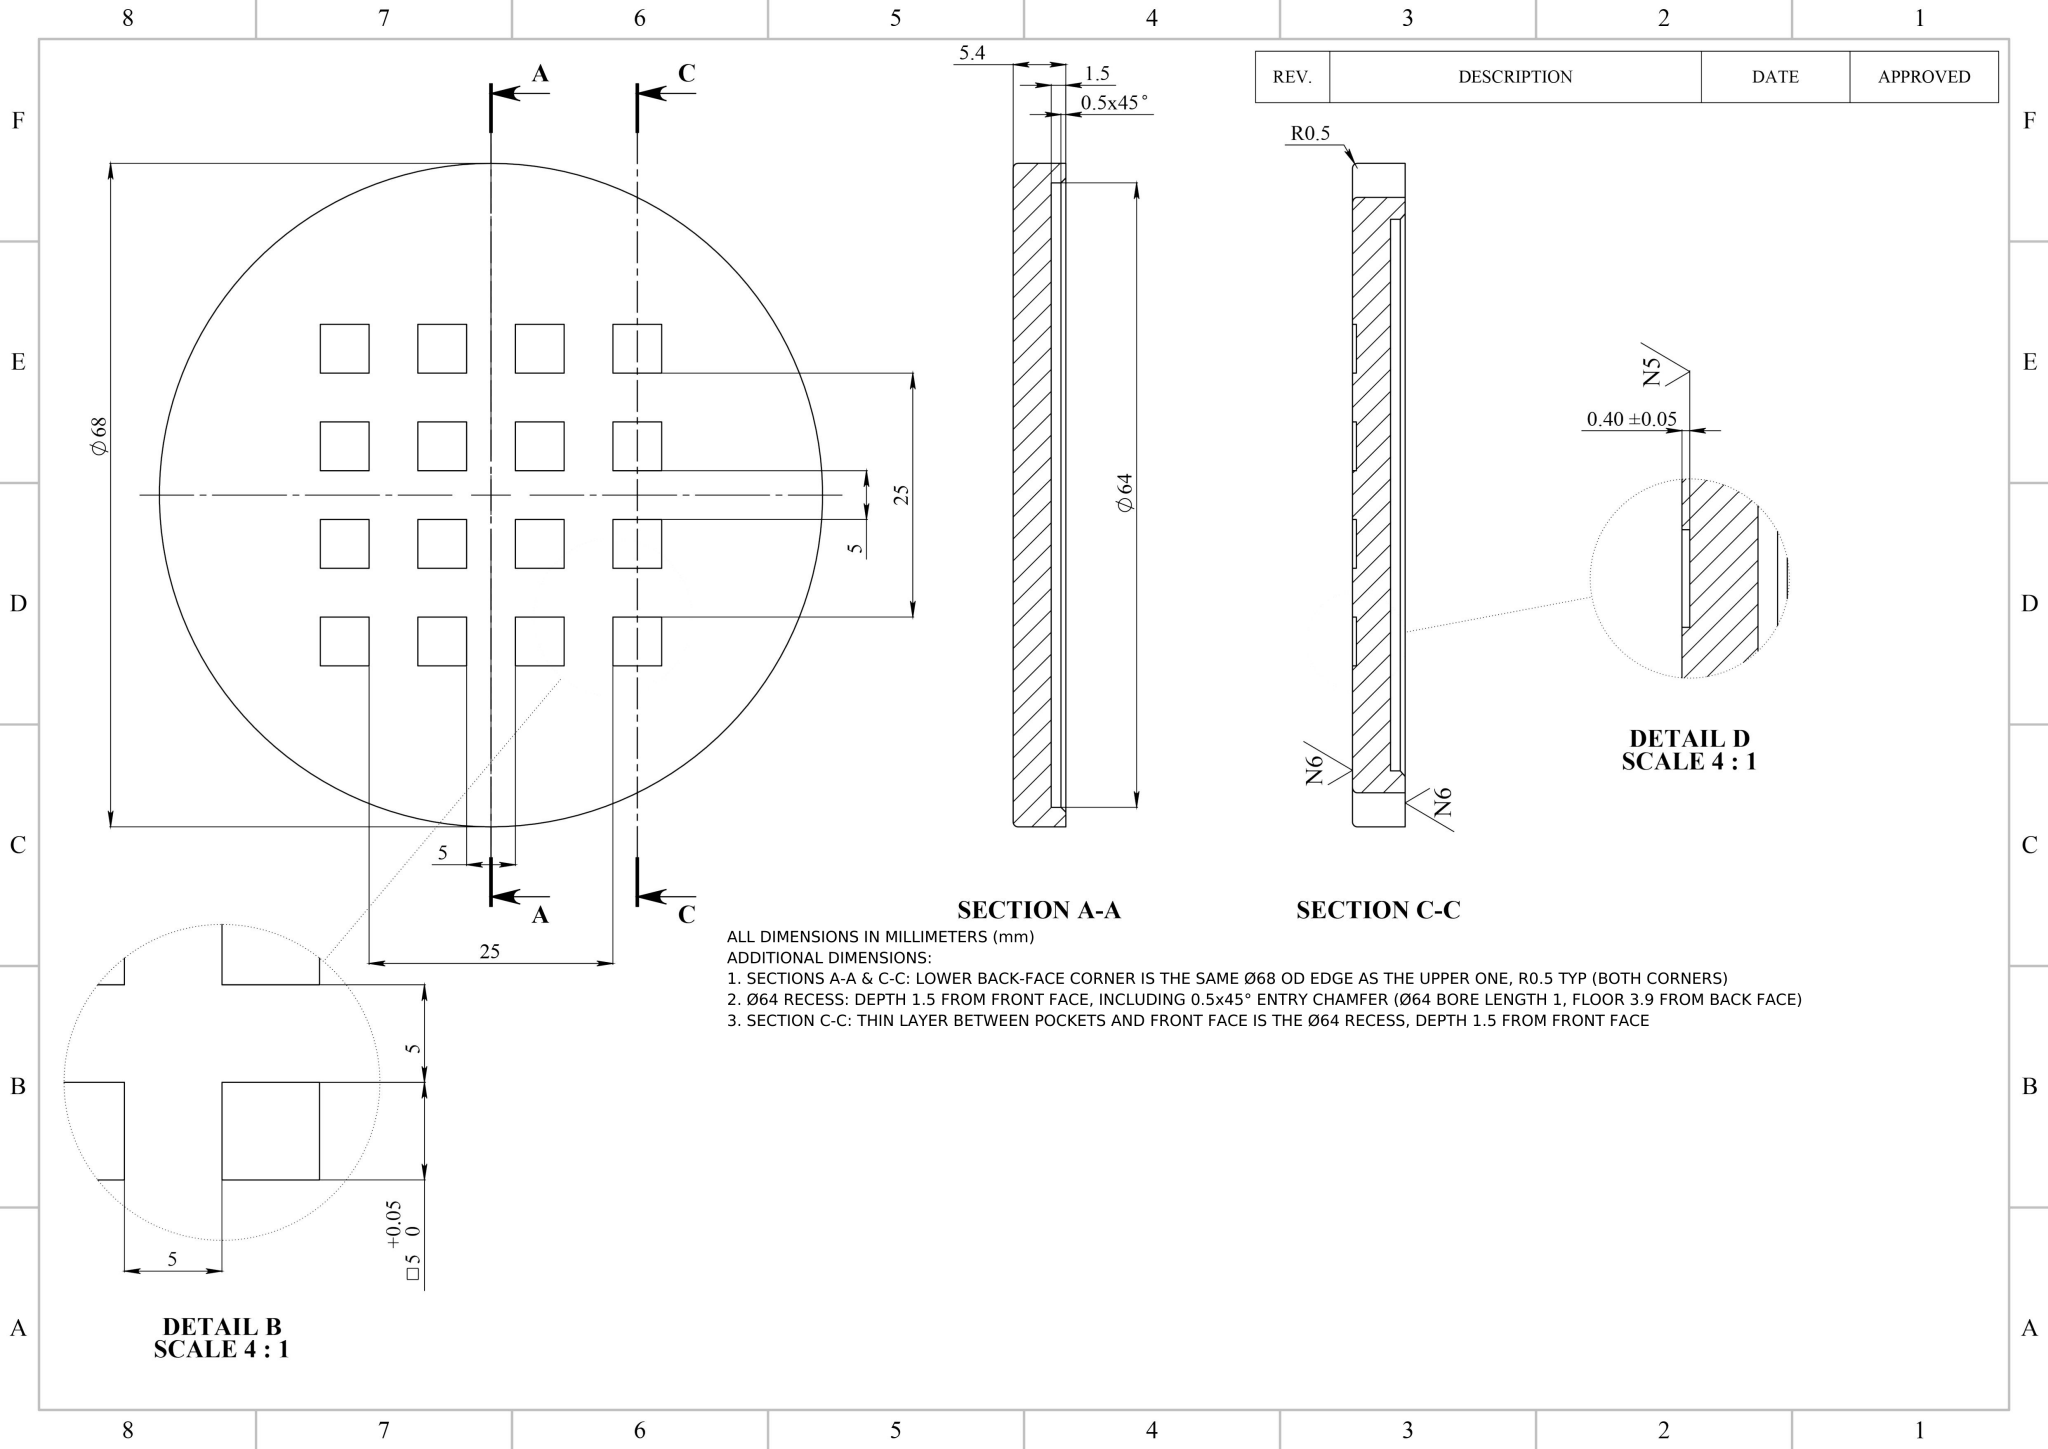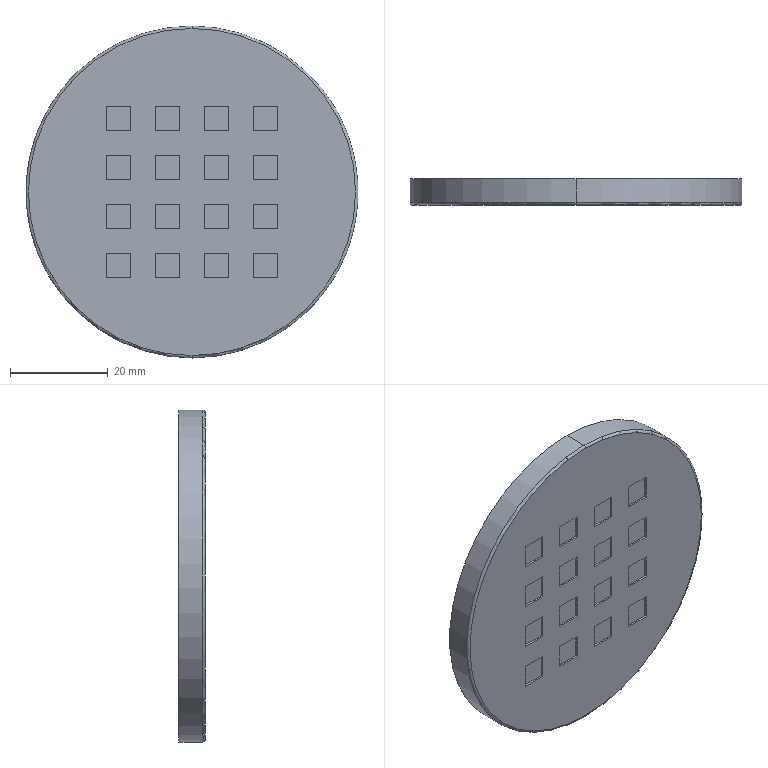Part | NX | mm | 1 solid | 91 faces | box 68 x 5.4 x 68 mm | volume 14589 mm3 | plane 83 | cylinder 4 | torus 2 | cone 2 | commonest cylinder face diameters 64 x2 68 x2